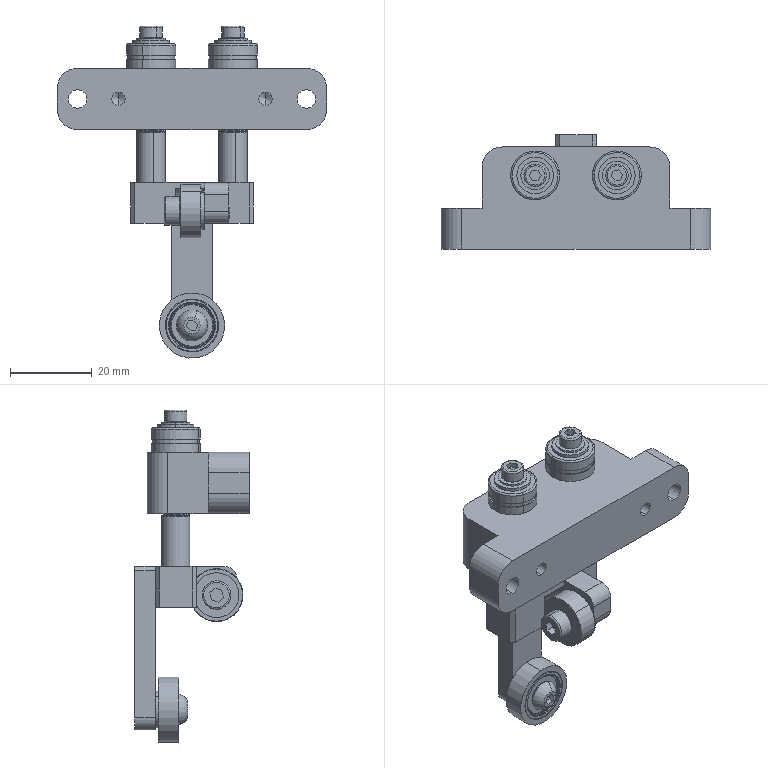Assembly | SolidWorks | mm | 22 component files | 22 solids | 500 faces | box 66 x 28 x 81.3 mm | volume 28584 mm3 | cylinder 181 | plane 159 | cone 82 | spline 50 | torus 28 | commonest cylinder face diameters 6 x24 12 x16 3 x16 4 x12 7 x10 11.5 x8 5.5 x8 4.3 x8
Bill of materials:
CoatedBearingMisumiUMBGW4-16 | 1 | 45 | Short annular cylinder with a central through bore. The face has several concentric recessed rings, so it looks like an outer ring, an inner ring and a recessed shield or seal face between them. Overall it looks like a shielded ball bearing.
DeepGrooveBallBearing624-2Z | 1 |  | Thick ring or short tube with a central through bore and flat end faces. One end face has a faint concentric line near the outer edge and another near the bore.
FlatWasher3 | 2 |  | Thin flat annular disc (looks like a plain washer) with a central round through hole and parallel flat faces.
FlatWasher4 | 4 |  | Thin flat annular disc (looks like a plain washer) with a central round through hole. It looks a little thicker relative to its diameter than unnamed part.
LinearBearingMisumiLMU6 | 2 | 45 | Cylindrical sleeve with a large central through bore. Two shallow circumferential grooves sit near the ends of the outer surface, and the end edges are rounded or chamfered. It looks like a linear-bushing-style sleeve.
SocketFlatHeadCapScrewM4_10 | 1 |  | Fastener-like part with a domed, button-style head and a plain cylindrical shank with a chamfered tip. The isometric view shows a hexagonal recess in the head.
SocketHeadCapScrew_M3_10 | 4 |  | Headed pin or screw-like part with a short cylindrical head and a smooth, longer cylindrical shank. The shank end and the head edges are chamfered or rounded.
SocketHeadCapScrew_M4_12 | 1 |  | Headed cylindrical part with a short cylindrical head and a smooth shank with a chamfered end. It is similar to unnamed part but has a shorter shank relative to the head.
SpringYIHEDAYVUR-D6-L15 | 2 | 45 | Thin-walled cylindrical tube, open at both ends. A thin rim or lip at one end shows a visible overlap or step, which makes it look like a wrapped or split sleeve.
WZH-20190520-F210StopBlockSeat | 1 | 45 | Elongated block-style bracket. A taller central section has two large parallel through bores, and lower end lugs extend on each side. Each end lug has a small horizontal through hole, and there are two small blind holes on the same long face.
WZH-20190520-F211StopBlockGuideRod | 2 | 45 | Slender cylindrical tube or pin with an axial bore and small chamfers at both ends.
WZH-20190520-F212StopBlockPusher | 1 | 45 | Compact bracket made of a T-shaped plate with two counterbored holes, a perpendicular downward arm with a round hole near its rounded end, and a side lug with a transverse hole.
Mates:
1. coincident | WZH-20190520-F210StopBlockSeat-1 plane at (0, 0, 0) dir (0, 0, 1) | assembly plane at (0, 0, 0) dir (0, 0, 1)
2. coincident | WZH-20190520-F210StopBlockSeat-1 plane at (0, 0, 0) dir (0, 1, 0) | assembly plane at (0, 0, 0) dir (0, 1, 0)
3. coincident | WZH-20190520-F210StopBlockSeat-1 plane at (0, 0, 0) dir (1, 0, 0) | assembly plane at (0, 0, 0) dir (1, 0, 0)
4. concentric | WZH-20190520-F210StopBlockSeat-1 face at (-10, 5.5, -24.471) dir (0, 0, 1) r 6 | LinearBearingMisumiLMU6-1 face at (-10, 5.5, 13.5) dir (0, 0, -1) r 6
5. coincident | WZH-20190520-F210StopBlockSeat-1 face at (0, 0, -5.5) dir (0, 0, 1) | LinearBearingMisumiLMU6-1 face at (-4.72, 3.634, -5.5) dir (0, 0, -1)
6. concentric | WZH-20190520-F210StopBlockSeat-1 face at (10, 5.5, -24.471) dir (0, 0, 1) r 6 | LinearBearingMisumiLMU6-2 face at (10, 5.5, 13.5) dir (0, 0, -1) r 6
7. coincident | WZH-20190520-F210StopBlockSeat-1 face at (0, 0, -5.5) dir (0, 0, 1) | LinearBearingMisumiLMU6-2 face at (10.33, 11.09, -5.5) dir (0, 0, -1)
8. concentric | LinearBearingMisumiLMU6-1 face at (-10, 5.5, 13.5) dir (0, 0, -1) r 3 | WZH-20190520-F211StopBlockGuideRod-1 face at (-10, 5.5, 13.554) dir (0, 0, -1) r 3
9. concentric | LinearBearingMisumiLMU6-2 face at (10, 5.5, 13.5) dir (0, 0, -1) r 3 | WZH-20190520-F211StopBlockGuideRod-2 face at (10, 5.5, 13.554) dir (0, 0, -1) r 3
10. concentric | WZH-20190520-F211StopBlockGuideRod-1 face at (-10, 5.5, 13.554) dir (0, 0, -1) r 3 | WZH-20190520-F212StopBlockPusher-1 face at (-10, 5.5, -23.446) dir (0, 0, 1) r 3
11. coincident | WZH-20190520-F211StopBlockGuideRod-1 face at (-10, 5.5, -23.446) dir (0, 0, -1) | WZH-20190520-F212StopBlockPusher-1 face at (-10, 5.5, -23.446) dir (0, 0, 1)
12. concentric | WZH-20190520-F211StopBlockGuideRod-2 face at (10, 5.5, 13.554) dir (0, 0, -1) r 3 | WZH-20190520-F212StopBlockPusher-1 face at (10, 5.5, -23.446) dir (0, 0, 1) r 3
13. coincident | WZH-20190520-F211StopBlockGuideRod-2 face at (10, 5.5, -23.446) dir (0, 0, -1) | WZH-20190520-F212StopBlockPusher-1 face at (10, 5.5, -23.446) dir (0, 0, 1)
14. concentric | WZH-20190520-F212StopBlockPusher-1 face at (3, -4.5, -27.446) dir (-1, 0, 0) r 2 | DeepGrooveBallBearing624-2Z-1 face at (-0.3, -4.5, -27.446) dir (-1, 0, 0) r 2
15. distance | WZH-20190520-F212StopBlockPusher-1 face at (3, -9.5, -30.446) dir (-1, 0, 0) | DeepGrooveBallBearing624-2Z-1 face at (2.2, -2.258, -25.453) dir (1, 0, 0)
16. distance | WZH-20190520-F211StopBlockGuideRod-1 face at (-10, 5.5, 13.554) dir (0, 0, 1) | LinearBearingMisumiLMU6-1 face at (-7.171, 4.5, 13.5) dir (0, 0, 1)
17. concentric | WZH-20190520-F211StopBlockGuideRod-1 face at (-10, 5.5, 13.554) dir (0, 0, -1) r 3 | SpringYIHEDAYVUR-D6-L15-1 face at (-10, 5.5, -21.95) dir (0, 0, 1) r 3.5
18. tangent | WZH-20190520-F210StopBlockSeat-1 face at (0, 0, -7.5) dir (0, 0, -1) | SpringYIHEDAYVUR-D6-L15-1 face at (-6.68, 6.009, -7.975) dir (1, 0, 0)
19. concentric | WZH-20190520-F211StopBlockGuideRod-2 face at (10, 5.5, 13.554) dir (0, 0, -1) r 3 | SpringYIHEDAYVUR-D6-L15-3 face at (10, 5.5, -21.95) dir (0, 0, 1) r 3.5
20. tangent | WZH-20190520-F210StopBlockSeat-1 face at (0, 0, -7.5) dir (0, 0, -1) | SpringYIHEDAYVUR-D6-L15-3 face at (13.317, 6.029, -7.975) dir (1, 0, 0)
21. concentric | WZH-20190520-F212StopBlockPusher-1 face at (-10, 5.5, -60.446) dir (0, 0, 1) r 1.7 | SocketHeadCapScrew_M3_10-4 face at (-10, 5.5, -30.39) dir (0, 0, -1) r 1.5
22. coincident | WZH-20190520-F212StopBlockPusher-1 face at (-10, 5.5, -27.046) dir (0, 0, -1) | SocketHeadCapScrew_M3_10-4 face at (-7.416, 4.56, -27.046) dir (0, 0, 1)
23. concentric | WZH-20190520-F212StopBlockPusher-1 face at (10, 5.5, -60.446) dir (0, 0, 1) r 1.7 | SocketHeadCapScrew_M3_10-1 face at (10, 5.5, -30.39) dir (0, 0, -1) r 1.5
24. coincident | WZH-20190520-F212StopBlockPusher-1 face at (10, 5.5, -27.046) dir (0, 0, -1) | SocketHeadCapScrew_M3_10-1 face at (12.749, 5.575, -27.046) dir (0, 0, 1)
25. coincident | WZH-20190520-F211StopBlockGuideRod-1 face at (-10, 5.5, 13.554) dir (0, 0, 1) | FlatWasher4-1 face at (-10, 5.5, 13.554) dir (0, 0, -1)
26. concentric | WZH-20190520-F211StopBlockGuideRod-1 face at (-10, 5.5, 13.554) dir (0, 0, -1) r 3 | FlatWasher4-1 face at (-10, 5.5, 14.354) dir (0, 0, -1) r 2.15
27. coincident | FlatWasher3-1 face at (-10, 5.5, 14.354) dir (0, 0, -1) | FlatWasher4-1 face at (-10, 5.5, 14.354) dir (0, 0, 1)
28. concentric | FlatWasher3-1 face at (-10, 5.5, 14.854) dir (0, 0, -1) r 1.6 | FlatWasher4-1 face at (-10, 5.5, 14.354) dir (0, 0, -1) r 2.15
29. concentric | WZH-20190520-F211StopBlockGuideRod-1 face at (-10, 5.5, 13.554) dir (0, 0, 1) r 1.5 | SocketHeadCapScrew_M3_10-3 face at (-10, 5.5, 18.198) dir (0, 0, 1) r 1.5
30. coincident | SocketHeadCapScrew_M3_10-3 face at (-7.638, 6.909, 14.854) dir (0, 0, -1) | FlatWasher3-1 face at (-10, 5.5, 14.854) dir (0, 0, 1)
31. coincident | WZH-20190520-F211StopBlockGuideRod-2 face at (10, 5.5, 13.554) dir (0, 0, 1) | FlatWasher4-2 face at (10, 5.5, 13.554) dir (0, 0, -1)
32. concentric | WZH-20190520-F211StopBlockGuideRod-2 face at (10, 5.5, 13.554) dir (0, 0, 1) r 1.5 | FlatWasher4-2 face at (10, 5.5, 14.354) dir (0, 0, -1) r 2.15
33. coincident | FlatWasher3-2 face at (10, 5.5, 14.354) dir (0, 0, -1) | FlatWasher4-2 face at (10, 5.5, 14.354) dir (0, 0, 1)
34. concentric | FlatWasher3-2 face at (10, 5.5, 14.854) dir (0, 0, -1) r 1.6 | FlatWasher4-2 face at (10, 5.5, 14.354) dir (0, 0, -1) r 2.15
35. concentric | WZH-20190520-F211StopBlockGuideRod-2 face at (10, 5.5, 13.554) dir (0, 0, 1) r 1.5 | SocketHeadCapScrew_M3_10-2 face at (10, 5.5, 18.198) dir (0, 0, 1) r 1.5
36. coincident | SocketHeadCapScrew_M3_10-2 face at (12.06, 7.322, 14.854) dir (0, 0, -1) | FlatWasher3-2 face at (10, 5.5, 14.854) dir (0, 0, 1)
37. coincident | WZH-20190520-F212StopBlockPusher-1 face at (0, 10.5, -25.446) dir (0, -1, 0) | FlatWasher4-3 face at (0, 10.5, -55.446) dir (0, 1, 0)
38. concentric | WZH-20190520-F212StopBlockPusher-1 face at (0, 15.5, -55.446) dir (0, 1, 0) r 2 | FlatWasher4-3 face at (0, 10.5, -55.446) dir (0, -1, 0) r 4.5
39. coincident | WZH-20190520-F212StopBlockPusher-1 face at (3, -9.5, -30.446) dir (-1, 0, 0) | FlatWasher4-4 face at (3, -4.5, -27.446) dir (1, 0, 0)
40. concentric | WZH-20190520-F212StopBlockPusher-1 face at (3, -4.5, -27.446) dir (-1, 0, 0) r 2 | FlatWasher4-4 face at (3, -4.5, -27.446) dir (-1, 0, 0) r 4.5
41. concentric | DeepGrooveBallBearing624-2Z-1 face at (-0.3, -4.5, -27.446) dir (-1, 0, 0) r 2 | SocketHeadCapScrew_M4_12-1 face at (-7.144, -4.5, -27.446) dir (-1, 0, 0) r 2
42. concentric | WZH-20190520-F212StopBlockPusher-1 face at (0, 15.5, -55.446) dir (0, 1, 0) r 2 | SocketFlatHeadCapScrewM4_10-2 face at (0, 2.5, -55.446) dir (0, 1, 0) r 2
43. concentric | WZH-20190520-F212StopBlockPusher-1 face at (0, 15.5, -55.446) dir (0, 1, 0) r 2 | CoatedBearingMisumiUMBGW4-16-1 face at (0, 57.2, -55.446) dir (0, -1, 0) r 2
44. coincident | FlatWasher4-3 face at (0, 9.7, -55.446) dir (0, -1, 0) | CoatedBearingMisumiUMBGW4-16-1 face at (-2.18, 9.7, -55.74) dir (0, 1, 0)
45. coincident | SocketFlatHeadCapScrewM4_10-2 face at (-3.571, 4.7, -54.148) dir (0, 1, 0) | CoatedBearingMisumiUMBGW4-16-1 face at (-3.072, 4.7, -55.86) dir (0, -1, 0)
46. coincident | DeepGrooveBallBearing624-2Z-1 face at (-2.8, -2.258, -25.453) dir (-1, 0, 0) | SocketHeadCapScrew_M4_12-1 face at (-2.8, -1.081, -28.196) dir (1, 0, 0)